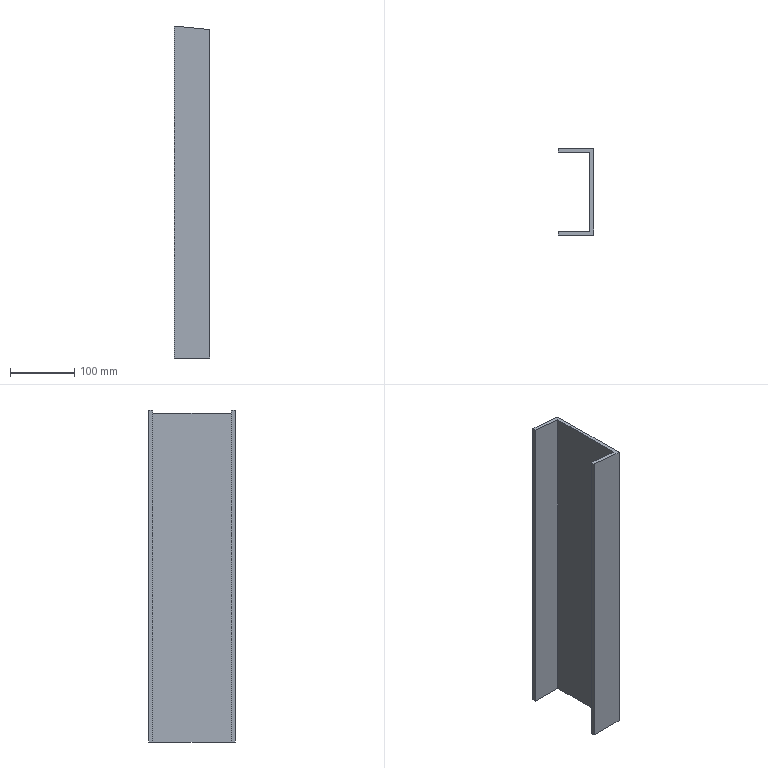Component | NX | LEFT_FRAME600_2 | 1 solid | 10 faces | box 55 x 135 x 517.27 mm | volume 717504 mm3 | plane 10
STEP:
#1=CARTESIAN_POINT('',(0.,0.,0.));
#2=DIRECTION('',(0.,0.,1.));
#3=DIRECTION('',(1.,0.,0.));
#4=AXIS2_PLACEMENT_3D('',#1,#2,#3);
#5=CARTESIAN_POINT('',(55.,0.,511.782));
#6=VERTEX_POINT('',#5);
#7=CARTESIAN_POINT('',(55.,135.,511.782));
#8=VERTEX_POINT('',#7);
#9=CARTESIAN_POINT('',(55.,135.,511.782));
#10=DIRECTION('',(0.,1.,-0.));
#11=VECTOR('',#10,1.);
#12=LINE('',#9,#11);
#13=CARTESIAN_POINT('',(55.,135.,530.));
#14=DIRECTION('',(1.,-0.,0.));
#15=DIRECTION('',(0.,1.,0.));
#16=AXIS2_PLACEMENT_3D('',#13,#14,#15);
#17=PLANE('',#16);
#18=CARTESIAN_POINT('',(0.,-18.218));
#19=DIRECTION('',(1.,-0.));
#20=VECTOR('',#19,1.);
#21=LINE('',#18,#20);
#22=(GEOMETRIC_REPRESENTATION_CONTEXT(2)PARAMETRIC_REPRESENTATION_CONTEXT()REPRESENTATION_CONTEXT('',''));
#23=DEFINITIONAL_REPRESENTATION('',(#21),#22);
#24=PCURVE('',#17,#23);
#25=CARTESIAN_POINT('',(96.917,-235.,507.598));
#26=DIRECTION('',(-0.09932,0.,-0.9951));
#27=DIRECTION('',(0.9951,0.,-0.09932));
#28=AXIS2_PLACEMENT_3D('',#25,#26,#27);
#29=PLANE('',#28);
#30=CARTESIAN_POINT('',(-42.125,-370.));
#31=DIRECTION('',(0.,-1.));
#32=VECTOR('',#31,1.);
#33=LINE('',#30,#32);
#34=(GEOMETRIC_REPRESENTATION_CONTEXT(2)PARAMETRIC_REPRESENTATION_CONTEXT()REPRESENTATION_CONTEXT('',''));
#35=DEFINITIONAL_REPRESENTATION('',(#33),#34);
#36=PCURVE('',#29,#35);
#37=SURFACE_CURVE('',#12,(#24,#36),.PCURVE_S1.);
#38=EDGE_CURVE('',#6,#8,#37,.T.);
#39=ORIENTED_EDGE('',*,*,#38,.F.);
#40=CARTESIAN_POINT('',(55.,0.,0.));
#41=VERTEX_POINT('',#40);
#42=CARTESIAN_POINT('',(55.,0.,530.));
#43=DIRECTION('',(0.,0.,-1.));
#44=VECTOR('',#43,1.);
#45=LINE('',#42,#44);
#46=CARTESIAN_POINT('',(-135.,0.));
#47=DIRECTION('',(0.,-1.));
#48=VECTOR('',#47,1.);
#49=LINE('',#46,#48);
#50=(GEOMETRIC_REPRESENTATION_CONTEXT(2)PARAMETRIC_REPRESENTATION_CONTEXT()REPRESENTATION_CONTEXT('',''));
#51=DEFINITIONAL_REPRESENTATION('',(#49),#50);
#52=PCURVE('',#17,#51);
#53=CARTESIAN_POINT('',(55.,0.,530.));
#54=DIRECTION('',(0.,-1.,0.));
#55=DIRECTION('',(0.,0.,1.));
#56=AXIS2_PLACEMENT_3D('',#53,#54,#55);
#57=PLANE('',#56);
#58=CARTESIAN_POINT('',(0.,0.));
#59=DIRECTION('',(-1.,0.));
#60=VECTOR('',#59,1.);
#61=LINE('',#58,#60);
#62=(GEOMETRIC_REPRESENTATION_CONTEXT(2)PARAMETRIC_REPRESENTATION_CONTEXT()REPRESENTATION_CONTEXT('',''));
#63=DEFINITIONAL_REPRESENTATION('',(#61),#62);
#64=PCURVE('',#57,#63);
#65=SURFACE_CURVE('',#45,(#52,#64),.PCURVE_S1.);
#66=EDGE_CURVE('',#6,#41,#65,.T.);
#67=ORIENTED_EDGE('',*,*,#66,.T.);
#68=CARTESIAN_POINT('',(55.,135.,0.));
#69=VERTEX_POINT('',#68);
#70=CARTESIAN_POINT('',(55.,135.,0.));
#71=DIRECTION('',(-0.,-1.,0.));
#72=VECTOR('',#71,1.);
#73=LINE('',#70,#72);
#74=CARTESIAN_POINT('',(0.,-530.));
#75=DIRECTION('',(-1.,0.));
#76=VECTOR('',#75,1.);
#77=LINE('',#74,#76);
#78=(GEOMETRIC_REPRESENTATION_CONTEXT(2)PARAMETRIC_REPRESENTATION_CONTEXT()REPRESENTATION_CONTEXT('',''));
#79=DEFINITIONAL_REPRESENTATION('',(#77),#78);
#80=PCURVE('',#17,#79);
#81=CARTESIAN_POINT('',(55.,0.,0.));
#82=DIRECTION('',(0.,0.,-1.));
#83=DIRECTION('',(1.,0.,0.));
#84=AXIS2_PLACEMENT_3D('',#81,#82,#83);
#85=PLANE('',#84);
#86=CARTESIAN_POINT('',(0.,-135.));
#87=DIRECTION('',(-0.,1.));
#88=VECTOR('',#87,1.);
#89=LINE('',#86,#88);
#90=(GEOMETRIC_REPRESENTATION_CONTEXT(2)PARAMETRIC_REPRESENTATION_CONTEXT()REPRESENTATION_CONTEXT('',''));
#91=DEFINITIONAL_REPRESENTATION('',(#89),#90);
#92=PCURVE('',#85,#91);
#93=SURFACE_CURVE('',#73,(#80,#92),.PCURVE_S1.);
#94=EDGE_CURVE('',#69,#41,#93,.T.);
#95=ORIENTED_EDGE('',*,*,#94,.F.);
#96=CARTESIAN_POINT('',(55.,135.,530.));
#97=DIRECTION('',(0.,0.,-1.));
#98=VECTOR('',#97,1.);
#99=LINE('',#96,#98);
#100=CARTESIAN_POINT('',(0.,0.));
#101=DIRECTION('',(0.,-1.));
#102=VECTOR('',#101,1.);
#103=LINE('',#100,#102);
#104=(GEOMETRIC_REPRESENTATION_CONTEXT(2)PARAMETRIC_REPRESENTATION_CONTEXT()REPRESENTATION_CONTEXT('',''));
#105=DEFINITIONAL_REPRESENTATION('',(#103),#104);
#106=PCURVE('',#17,#105);
#107=CARTESIAN_POINT('',(0.,135.,530.));
#108=DIRECTION('',(0.,1.,0.));
#109=DIRECTION('',(0.,0.,-1.));
#110=AXIS2_PLACEMENT_3D('',#107,#108,#109);
#111=PLANE('',#110);
#112=CARTESIAN_POINT('',(0.,-55.));
#113=DIRECTION('',(1.,0.));
#114=VECTOR('',#113,1.);
#115=LINE('',#112,#114);
#116=(GEOMETRIC_REPRESENTATION_CONTEXT(2)PARAMETRIC_REPRESENTATION_CONTEXT()REPRESENTATION_CONTEXT('',''));
#117=DEFINITIONAL_REPRESENTATION('',(#115),#116);
#118=PCURVE('',#111,#117);
#119=SURFACE_CURVE('',#99,(#106,#118),.PCURVE_S1.);
#120=EDGE_CURVE('',#8,#69,#119,.T.);
#121=ORIENTED_EDGE('',*,*,#120,.F.);
#122=EDGE_LOOP('',(#39,#67,#95,#121));
#123=FACE_BOUND('',#122,.T.);
#124=ADVANCED_FACE('',(#123),#17,.T.);
#125=CARTESIAN_POINT('',(0.,0.,517.272));
#126=VERTEX_POINT('',#125);
#127=CARTESIAN_POINT('',(53.2,0.,511.962));
#128=DIRECTION('',(0.9951,0.,-0.09932));
#129=VECTOR('',#128,1.);
#130=LINE('',#127,#129);
#131=CARTESIAN_POINT('',(-18.038,1.8));
#132=DIRECTION('',(-0.09932,-0.9951));
#133=VECTOR('',#132,1.);
#134=LINE('',#131,#133);
#135=(GEOMETRIC_REPRESENTATION_CONTEXT(2)PARAMETRIC_REPRESENTATION_CONTEXT()REPRESENTATION_CONTEXT('',''));
#136=DEFINITIONAL_REPRESENTATION('',(#134),#135);
#137=PCURVE('',#57,#136);
#138=CARTESIAN_POINT('',(-43.934,-235.));
#139=DIRECTION('',(1.,0.));
#140=VECTOR('',#139,1.);
#141=LINE('',#138,#140);
#142=(GEOMETRIC_REPRESENTATION_CONTEXT(2)PARAMETRIC_REPRESENTATION_CONTEXT()REPRESENTATION_CONTEXT('',''));
#143=DEFINITIONAL_REPRESENTATION('',(#141),#142);
#144=PCURVE('',#29,#143);
#145=SURFACE_CURVE('',#130,(#137,#144),.PCURVE_S1.);
#146=EDGE_CURVE('',#126,#6,#145,.T.);
#147=ORIENTED_EDGE('',*,*,#146,.F.);
#148=CARTESIAN_POINT('',(0.,0.,0.));
#149=VERTEX_POINT('',#148);
#150=CARTESIAN_POINT('',(0.,0.,530.));
#151=DIRECTION('',(0.,0.,-1.));
#152=VECTOR('',#151,1.);
#153=LINE('',#150,#152);
#154=CARTESIAN_POINT('',(0.,55.));
#155=DIRECTION('',(-1.,0.));
#156=VECTOR('',#155,1.);
#157=LINE('',#154,#156);
#158=(GEOMETRIC_REPRESENTATION_CONTEXT(2)PARAMETRIC_REPRESENTATION_CONTEXT()REPRESENTATION_CONTEXT('',''));
#159=DEFINITIONAL_REPRESENTATION('',(#157),#158);
#160=PCURVE('',#57,#159);
#161=CARTESIAN_POINT('',(0.,0.,530.));
#162=DIRECTION('',(-1.,0.,0.));
#163=DIRECTION('',(-0.,-1.,0.));
#164=AXIS2_PLACEMENT_3D('',#161,#162,#163);
#165=PLANE('',#164);
#166=CARTESIAN_POINT('',(0.,0.));
#167=DIRECTION('',(0.,-1.));
#168=VECTOR('',#167,1.);
#169=LINE('',#166,#168);
#170=(GEOMETRIC_REPRESENTATION_CONTEXT(2)PARAMETRIC_REPRESENTATION_CONTEXT()REPRESENTATION_CONTEXT('',''));
#171=DEFINITIONAL_REPRESENTATION('',(#169),#170);
#172=PCURVE('',#165,#171);
#173=SURFACE_CURVE('',#153,(#160,#172),.PCURVE_S1.);
#174=EDGE_CURVE('',#126,#149,#173,.T.);
#175=ORIENTED_EDGE('',*,*,#174,.T.);
#176=CARTESIAN_POINT('',(55.,0.,0.));
#177=DIRECTION('',(-1.,0.,0.));
#178=VECTOR('',#177,1.);
#179=LINE('',#176,#178);
#180=CARTESIAN_POINT('',(-530.,0.));
#181=DIRECTION('',(0.,1.));
#182=VECTOR('',#181,1.);
#183=LINE('',#180,#182);
#184=(GEOMETRIC_REPRESENTATION_CONTEXT(2)PARAMETRIC_REPRESENTATION_CONTEXT()REPRESENTATION_CONTEXT('',''));
#185=DEFINITIONAL_REPRESENTATION('',(#183),#184);
#186=PCURVE('',#57,#185);
#187=CARTESIAN_POINT('',(0.,0.));
#188=DIRECTION('',(-1.,0.));
#189=VECTOR('',#188,1.);
#190=LINE('',#187,#189);
#191=(GEOMETRIC_REPRESENTATION_CONTEXT(2)PARAMETRIC_REPRESENTATION_CONTEXT()REPRESENTATION_CONTEXT('',''));
#192=DEFINITIONAL_REPRESENTATION('',(#190),#191);
#193=PCURVE('',#85,#192);
#194=SURFACE_CURVE('',#179,(#186,#193),.PCURVE_S1.);
#195=EDGE_CURVE('',#41,#149,#194,.T.);
#196=ORIENTED_EDGE('',*,*,#195,.F.);
#197=ORIENTED_EDGE('',*,*,#66,.F.);
#198=EDGE_LOOP('',(#147,#175,#196,#197));
#199=FACE_BOUND('',#198,.T.);
#200=ADVANCED_FACE('',(#199),#57,.T.);
#201=CARTESIAN_POINT('',(0.,6.,517.272));
#202=VERTEX_POINT('',#201);
#203=CARTESIAN_POINT('',(0.,0.,517.272));
#204=DIRECTION('',(-0.,-1.,0.));
#205=VECTOR('',#204,1.);
#206=LINE('',#203,#205);
#207=CARTESIAN_POINT('',(0.,-12.728));
#208=DIRECTION('',(1.,0.));
#209=VECTOR('',#208,1.);
#210=LINE('',#207,#209);
#211=(GEOMETRIC_REPRESENTATION_CONTEXT(2)PARAMETRIC_REPRESENTATION_CONTEXT()REPRESENTATION_CONTEXT('',''));
#212=DEFINITIONAL_REPRESENTATION('',(#210),#211);
#213=PCURVE('',#165,#212);
#214=CARTESIAN_POINT('',(-97.398,-235.));
#215=DIRECTION('',(-0.,1.));
#216=VECTOR('',#215,1.);
#217=LINE('',#214,#216);
#218=(GEOMETRIC_REPRESENTATION_CONTEXT(2)PARAMETRIC_REPRESENTATION_CONTEXT()REPRESENTATION_CONTEXT('',''));
#219=DEFINITIONAL_REPRESENTATION('',(#217),#218);
#220=PCURVE('',#29,#219);
#221=SURFACE_CURVE('',#206,(#213,#220),.PCURVE_S1.);
#222=EDGE_CURVE('',#202,#126,#221,.T.);
#223=ORIENTED_EDGE('',*,*,#222,.F.);
#224=CARTESIAN_POINT('',(0.,6.,0.));
#225=VERTEX_POINT('',#224);
#226=CARTESIAN_POINT('',(0.,6.,530.));
#227=DIRECTION('',(0.,0.,-1.));
#228=VECTOR('',#227,1.);
#229=LINE('',#226,#228);
#230=CARTESIAN_POINT('',(-6.,0.));
#231=DIRECTION('',(0.,-1.));
#232=VECTOR('',#231,1.);
#233=LINE('',#230,#232);
#234=(GEOMETRIC_REPRESENTATION_CONTEXT(2)PARAMETRIC_REPRESENTATION_CONTEXT()REPRESENTATION_CONTEXT('',''));
#235=DEFINITIONAL_REPRESENTATION('',(#233),#234);
#236=PCURVE('',#165,#235);
#237=CARTESIAN_POINT('',(0.,6.,530.));
#238=DIRECTION('',(0.,1.,0.));
#239=DIRECTION('',(-1.,0.,0.));
#240=AXIS2_PLACEMENT_3D('',#237,#238,#239);
#241=PLANE('',#240);
#242=CARTESIAN_POINT('',(0.,0.));
#243=DIRECTION('',(0.,-1.));
#244=VECTOR('',#243,1.);
#245=LINE('',#242,#244);
#246=(GEOMETRIC_REPRESENTATION_CONTEXT(2)PARAMETRIC_REPRESENTATION_CONTEXT()REPRESENTATION_CONTEXT('',''));
#247=DEFINITIONAL_REPRESENTATION('',(#245),#246);
#248=PCURVE('',#241,#247);
#249=SURFACE_CURVE('',#229,(#236,#248),.PCURVE_S1.);
#250=EDGE_CURVE('',#202,#225,#249,.T.);
#251=ORIENTED_EDGE('',*,*,#250,.T.);
#252=CARTESIAN_POINT('',(0.,0.,0.));
#253=DIRECTION('',(0.,1.,0.));
#254=VECTOR('',#253,1.);
#255=LINE('',#252,#254);
#256=CARTESIAN_POINT('',(0.,-530.));
#257=DIRECTION('',(-1.,0.));
#258=VECTOR('',#257,1.);
#259=LINE('',#256,#258);
#260=(GEOMETRIC_REPRESENTATION_CONTEXT(2)PARAMETRIC_REPRESENTATION_CONTEXT()REPRESENTATION_CONTEXT('',''));
#261=DEFINITIONAL_REPRESENTATION('',(#259),#260);
#262=PCURVE('',#165,#261);
#263=CARTESIAN_POINT('',(-55.,0.));
#264=DIRECTION('',(0.,-1.));
#265=VECTOR('',#264,1.);
#266=LINE('',#263,#265);
#267=(GEOMETRIC_REPRESENTATION_CONTEXT(2)PARAMETRIC_REPRESENTATION_CONTEXT()REPRESENTATION_CONTEXT('',''));
#268=DEFINITIONAL_REPRESENTATION('',(#266),#267);
#269=PCURVE('',#85,#268);
#270=SURFACE_CURVE('',#255,(#262,#269),.PCURVE_S1.);
#271=EDGE_CURVE('',#149,#225,#270,.T.);
#272=ORIENTED_EDGE('',*,*,#271,.F.);
#273=ORIENTED_EDGE('',*,*,#174,.F.);
#274=EDGE_LOOP('',(#223,#251,#272,#273));
#275=FACE_BOUND('',#274,.T.);
#276=ADVANCED_FACE('',(#275),#165,.T.);
#277=CARTESIAN_POINT('',(49.,6.,512.381));
#278=VERTEX_POINT('',#277);
#279=CARTESIAN_POINT('',(-1.258,6.,517.397));
#280=DIRECTION('',(-0.9951,0.,0.09932));
#281=VECTOR('',#280,1.);
#282=LINE('',#279,#281);
#283=CARTESIAN_POINT('',(1.258,-12.603));
#284=DIRECTION('',(0.9951,0.09932));
#285=VECTOR('',#284,1.);
#286=LINE('',#283,#285);
#287=(GEOMETRIC_REPRESENTATION_CONTEXT(2)PARAMETRIC_REPRESENTATION_CONTEXT()REPRESENTATION_CONTEXT('',''));
#288=DEFINITIONAL_REPRESENTATION('',(#286),#287);
#289=PCURVE('',#241,#288);
#290=CARTESIAN_POINT('',(-98.662,-241.));
#291=DIRECTION('',(-1.,-0.));
#292=VECTOR('',#291,1.);
#293=LINE('',#290,#292);
#294=(GEOMETRIC_REPRESENTATION_CONTEXT(2)PARAMETRIC_REPRESENTATION_CONTEXT()REPRESENTATION_CONTEXT('',''));
#295=DEFINITIONAL_REPRESENTATION('',(#293),#294);
#296=PCURVE('',#29,#295);
#297=SURFACE_CURVE('',#282,(#289,#296),.PCURVE_S1.);
#298=EDGE_CURVE('',#278,#202,#297,.T.);
#299=ORIENTED_EDGE('',*,*,#298,.F.);
#300=CARTESIAN_POINT('',(49.,6.,0.));
#301=VERTEX_POINT('',#300);
#302=CARTESIAN_POINT('',(49.,6.,530.));
#303=DIRECTION('',(0.,0.,-1.));
#304=VECTOR('',#303,1.);
#305=LINE('',#302,#304);
#306=CARTESIAN_POINT('',(-49.,0.));
#307=DIRECTION('',(0.,-1.));
#308=VECTOR('',#307,1.);
#309=LINE('',#306,#308);
#310=(GEOMETRIC_REPRESENTATION_CONTEXT(2)PARAMETRIC_REPRESENTATION_CONTEXT()REPRESENTATION_CONTEXT('',''));
#311=DEFINITIONAL_REPRESENTATION('',(#309),#310);
#312=PCURVE('',#241,#311);
#313=CARTESIAN_POINT('',(49.,6.,530.));
#314=DIRECTION('',(-1.,0.,0.));
#315=DIRECTION('',(-0.,-1.,0.));
#316=AXIS2_PLACEMENT_3D('',#313,#314,#315);
#317=PLANE('',#316);
#318=CARTESIAN_POINT('',(0.,0.));
#319=DIRECTION('',(0.,-1.));
#320=VECTOR('',#319,1.);
#321=LINE('',#318,#320);
#322=(GEOMETRIC_REPRESENTATION_CONTEXT(2)PARAMETRIC_REPRESENTATION_CONTEXT()REPRESENTATION_CONTEXT('',''));
#323=DEFINITIONAL_REPRESENTATION('',(#321),#322);
#324=PCURVE('',#317,#323);
#325=SURFACE_CURVE('',#305,(#312,#324),.PCURVE_S1.);
#326=EDGE_CURVE('',#278,#301,#325,.T.);
#327=ORIENTED_EDGE('',*,*,#326,.T.);
#328=CARTESIAN_POINT('',(0.,6.,0.));
#329=DIRECTION('',(1.,-0.,0.));
#330=VECTOR('',#329,1.);
#331=LINE('',#328,#330);
#332=CARTESIAN_POINT('',(0.,-530.));
#333=DIRECTION('',(-1.,0.));
#334=VECTOR('',#333,1.);
#335=LINE('',#332,#334);
#336=(GEOMETRIC_REPRESENTATION_CONTEXT(2)PARAMETRIC_REPRESENTATION_CONTEXT()REPRESENTATION_CONTEXT('',''));
#337=DEFINITIONAL_REPRESENTATION('',(#335),#336);
#338=PCURVE('',#241,#337);
#339=CARTESIAN_POINT('',(-55.,-6.));
#340=DIRECTION('',(1.,0.));
#341=VECTOR('',#340,1.);
#342=LINE('',#339,#341);
#343=(GEOMETRIC_REPRESENTATION_CONTEXT(2)PARAMETRIC_REPRESENTATION_CONTEXT()REPRESENTATION_CONTEXT('',''));
#344=DEFINITIONAL_REPRESENTATION('',(#342),#343);
#345=PCURVE('',#85,#344);
#346=SURFACE_CURVE('',#331,(#338,#345),.PCURVE_S1.);
#347=EDGE_CURVE('',#225,#301,#346,.T.);
#348=ORIENTED_EDGE('',*,*,#347,.F.);
#349=ORIENTED_EDGE('',*,*,#250,.F.);
#350=EDGE_LOOP('',(#299,#327,#348,#349));
#351=FACE_BOUND('',#350,.T.);
#352=ADVANCED_FACE('',(#351),#241,.T.);
#353=CARTESIAN_POINT('',(49.,129.,512.381));
#354=VERTEX_POINT('',#353);
#355=CARTESIAN_POINT('',(49.,6.,512.381));
#356=DIRECTION('',(-0.,-1.,0.));
#357=VECTOR('',#356,1.);
#358=LINE('',#355,#357);
#359=CARTESIAN_POINT('',(0.,-17.619));
#360=DIRECTION('',(1.,0.));
#361=VECTOR('',#360,1.);
#362=LINE('',#359,#361);
#363=(GEOMETRIC_REPRESENTATION_CONTEXT(2)PARAMETRIC_REPRESENTATION_CONTEXT()REPRESENTATION_CONTEXT('',''));
#364=DEFINITIONAL_REPRESENTATION('',(#362),#363);
#365=PCURVE('',#317,#364);
#366=CARTESIAN_POINT('',(-48.155,-241.));
#367=DIRECTION('',(-0.,1.));
#368=VECTOR('',#367,1.);
#369=LINE('',#366,#368);
#370=(GEOMETRIC_REPRESENTATION_CONTEXT(2)PARAMETRIC_REPRESENTATION_CONTEXT()REPRESENTATION_CONTEXT('',''));
#371=DEFINITIONAL_REPRESENTATION('',(#369),#370);
#372=PCURVE('',#29,#371);
#373=SURFACE_CURVE('',#358,(#365,#372),.PCURVE_S1.);
#374=EDGE_CURVE('',#354,#278,#373,.T.);
#375=ORIENTED_EDGE('',*,*,#374,.F.);
#376=CARTESIAN_POINT('',(49.,129.,0.));
#377=VERTEX_POINT('',#376);
#378=CARTESIAN_POINT('',(49.,129.,530.));
#379=DIRECTION('',(0.,0.,-1.));
#380=VECTOR('',#379,1.);
#381=LINE('',#378,#380);
#382=CARTESIAN_POINT('',(-123.,0.));
#383=DIRECTION('',(0.,-1.));
#384=VECTOR('',#383,1.);
#385=LINE('',#382,#384);
#386=(GEOMETRIC_REPRESENTATION_CONTEXT(2)PARAMETRIC_REPRESENTATION_CONTEXT()REPRESENTATION_CONTEXT('',''));
#387=DEFINITIONAL_REPRESENTATION('',(#385),#386);
#388=PCURVE('',#317,#387);
#389=CARTESIAN_POINT('',(49.,129.,530.));
#390=DIRECTION('',(-0.,-1.,0.));
#391=DIRECTION('',(1.,-0.,0.));
#392=AXIS2_PLACEMENT_3D('',#389,#390,#391);
#393=PLANE('',#392);
#394=CARTESIAN_POINT('',(0.,0.));
#395=DIRECTION('',(0.,-1.));
#396=VECTOR('',#395,1.);
#397=LINE('',#394,#396);
#398=(GEOMETRIC_REPRESENTATION_CONTEXT(2)PARAMETRIC_REPRESENTATION_CONTEXT()REPRESENTATION_CONTEXT('',''));
#399=DEFINITIONAL_REPRESENTATION('',(#397),#398);
#400=PCURVE('',#393,#399);
#401=SURFACE_CURVE('',#381,(#388,#400),.PCURVE_S1.);
#402=EDGE_CURVE('',#354,#377,#401,.T.);
#403=ORIENTED_EDGE('',*,*,#402,.T.);
#404=CARTESIAN_POINT('',(49.,6.,0.));
#405=DIRECTION('',(0.,1.,0.));
#406=VECTOR('',#405,1.);
#407=LINE('',#404,#406);
#408=CARTESIAN_POINT('',(0.,-530.));
#409=DIRECTION('',(-1.,0.));
#410=VECTOR('',#409,1.);
#411=LINE('',#408,#410);
#412=(GEOMETRIC_REPRESENTATION_CONTEXT(2)PARAMETRIC_REPRESENTATION_CONTEXT()REPRESENTATION_CONTEXT('',''));
#413=DEFINITIONAL_REPRESENTATION('',(#411),#412);
#414=PCURVE('',#317,#413);
#415=CARTESIAN_POINT('',(-6.,-6.));
#416=DIRECTION('',(0.,-1.));
#417=VECTOR('',#416,1.);
#418=LINE('',#415,#417);
#419=(GEOMETRIC_REPRESENTATION_CONTEXT(2)PARAMETRIC_REPRESENTATION_CONTEXT()REPRESENTATION_CONTEXT('',''));
#420=DEFINITIONAL_REPRESENTATION('',(#418),#419);
#421=PCURVE('',#85,#420);
#422=SURFACE_CURVE('',#407,(#414,#421),.PCURVE_S1.);
#423=EDGE_CURVE('',#301,#377,#422,.T.);
#424=ORIENTED_EDGE('',*,*,#423,.F.);
#425=ORIENTED_EDGE('',*,*,#326,.F.);
#426=EDGE_LOOP('',(#375,#403,#424,#425));
#427=FACE_BOUND('',#426,.T.);
#428=ADVANCED_FACE('',(#427),#317,.T.);
#429=CARTESIAN_POINT('',(0.,129.,517.272));
#430=VERTEX_POINT('',#429);
#431=CARTESIAN_POINT('',(47.259,129.,512.555));
#432=DIRECTION('',(0.9951,-0.,-0.09932));
#433=VECTOR('',#432,1.);
#434=LINE('',#431,#433);
#435=CARTESIAN_POINT('',(-1.741,-17.445));
#436=DIRECTION('',(0.9951,-0.09932));
#437=VECTOR('',#436,1.);
#438=LINE('',#435,#437);
#439=(GEOMETRIC_REPRESENTATION_CONTEXT(2)PARAMETRIC_REPRESENTATION_CONTEXT()REPRESENTATION_CONTEXT('',''));
#440=DEFINITIONAL_REPRESENTATION('',(#438),#439);
#441=PCURVE('',#393,#440);
#442=CARTESIAN_POINT('',(-49.905,-364.));
#443=DIRECTION('',(1.,0.));
#444=VECTOR('',#443,1.);
#445=LINE('',#442,#444);
#446=(GEOMETRIC_REPRESENTATION_CONTEXT(2)PARAMETRIC_REPRESENTATION_CONTEXT()REPRESENTATION_CONTEXT('',''));
#447=DEFINITIONAL_REPRESENTATION('',(#445),#446);
#448=PCURVE('',#29,#447);
#449=SURFACE_CURVE('',#434,(#441,#448),.PCURVE_S1.);
#450=EDGE_CURVE('',#430,#354,#449,.T.);
#451=ORIENTED_EDGE('',*,*,#450,.F.);
#452=CARTESIAN_POINT('',(0.,129.,0.));
#453=VERTEX_POINT('',#452);
#454=CARTESIAN_POINT('',(0.,129.,530.));
#455=DIRECTION('',(0.,0.,-1.));
#456=VECTOR('',#455,1.);
#457=LINE('',#454,#456);
#458=CARTESIAN_POINT('',(-49.,0.));
#459=DIRECTION('',(0.,-1.));
#460=VECTOR('',#459,1.);
#461=LINE('',#458,#460);
#462=(GEOMETRIC_REPRESENTATION_CONTEXT(2)PARAMETRIC_REPRESENTATION_CONTEXT()REPRESENTATION_CONTEXT('',''));
#463=DEFINITIONAL_REPRESENTATION('',(#461),#462);
#464=PCURVE('',#393,#463);
#465=CARTESIAN_POINT('',(0.,129.,530.));
#466=DIRECTION('',(-1.,0.,0.));
#467=DIRECTION('',(0.,0.,-1.));
#468=AXIS2_PLACEMENT_3D('',#465,#466,#467);
#469=PLANE('',#468);
#470=CARTESIAN_POINT('',(0.,0.));
#471=DIRECTION('',(1.,0.));
#472=VECTOR('',#471,1.);
#473=LINE('',#470,#472);
#474=(GEOMETRIC_REPRESENTATION_CONTEXT(2)PARAMETRIC_REPRESENTATION_CONTEXT()REPRESENTATION_CONTEXT('',''));
#475=DEFINITIONAL_REPRESENTATION('',(#473),#474);
#476=PCURVE('',#469,#475);
#477=SURFACE_CURVE('',#457,(#464,#476),.PCURVE_S1.);
#478=EDGE_CURVE('',#430,#453,#477,.T.);
#479=ORIENTED_EDGE('',*,*,#478,.T.);
#480=CARTESIAN_POINT('',(49.,129.,0.));
#481=DIRECTION('',(-1.,0.,0.));
#482=VECTOR('',#481,1.);
#483=LINE('',#480,#482);
#484=CARTESIAN_POINT('',(0.,-530.));
#485=DIRECTION('',(-1.,0.));
#486=VECTOR('',#485,1.);
#487=LINE('',#484,#486);
#488=(GEOMETRIC_REPRESENTATION_CONTEXT(2)PARAMETRIC_REPRESENTATION_CONTEXT()REPRESENTATION_CONTEXT('',''));
#489=DEFINITIONAL_REPRESENTATION('',(#487),#488);
#490=PCURVE('',#393,#489);
#491=CARTESIAN_POINT('',(-6.,-129.));
#492=DIRECTION('',(-1.,-0.));
#493=VECTOR('',#492,1.);
#494=LINE('',#491,#493);
#495=(GEOMETRIC_REPRESENTATION_CONTEXT(2)PARAMETRIC_REPRESENTATION_CONTEXT()REPRESENTATION_CONTEXT('',''));
#496=DEFINITIONAL_REPRESENTATION('',(#494),#495);
#497=PCURVE('',#85,#496);
#498=SURFACE_CURVE('',#483,(#490,#497),.PCURVE_S1.);
#499=EDGE_CURVE('',#377,#453,#498,.T.);
#500=ORIENTED_EDGE('',*,*,#499,.F.);
#501=ORIENTED_EDGE('',*,*,#402,.F.);
#502=EDGE_LOOP('',(#451,#479,#500,#501));
#503=FACE_BOUND('',#502,.T.);
#504=ADVANCED_FACE('',(#503),#393,.T.);
#505=CARTESIAN_POINT('',(0.,135.,517.272));
#506=VERTEX_POINT('',#505);
#507=CARTESIAN_POINT('',(0.,129.,517.272));
#508=DIRECTION('',(0.,-1.,0.));
#509=VECTOR('',#508,1.);
#510=LINE('',#507,#509);
#511=CARTESIAN_POINT('',(12.728,0.));
#512=DIRECTION('',(0.,1.));
#513=VECTOR('',#512,1.);
#514=LINE('',#511,#513);
#515=(GEOMETRIC_REPRESENTATION_CONTEXT(2)PARAMETRIC_REPRESENTATION_CONTEXT()REPRESENTATION_CONTEXT('',''));
#516=DEFINITIONAL_REPRESENTATION('',(#514),#515);
#517=PCURVE('',#469,#516);
#518=CARTESIAN_POINT('',(-97.398,-364.));
#519=DIRECTION('',(0.,1.));
#520=VECTOR('',#519,1.);
#521=LINE('',#518,#520);
#522=(GEOMETRIC_REPRESENTATION_CONTEXT(2)PARAMETRIC_REPRESENTATION_CONTEXT()REPRESENTATION_CONTEXT('',''));
#523=DEFINITIONAL_REPRESENTATION('',(#521),#522);
#524=PCURVE('',#29,#523);
#525=SURFACE_CURVE('',#510,(#517,#524),.PCURVE_S1.);
#526=EDGE_CURVE('',#506,#430,#525,.T.);
#527=ORIENTED_EDGE('',*,*,#526,.F.);
#528=CARTESIAN_POINT('',(0.,135.,0.));
#529=VERTEX_POINT('',#528);
#530=CARTESIAN_POINT('',(0.,135.,530.));
#531=DIRECTION('',(0.,0.,-1.));
#532=VECTOR('',#531,1.);
#533=LINE('',#530,#532);
#534=CARTESIAN_POINT('',(0.,-6.));
#535=DIRECTION('',(1.,0.));
#536=VECTOR('',#535,1.);
#537=LINE('',#534,#536);
#538=(GEOMETRIC_REPRESENTATION_CONTEXT(2)PARAMETRIC_REPRESENTATION_CONTEXT()REPRESENTATION_CONTEXT('',''));
#539=DEFINITIONAL_REPRESENTATION('',(#537),#538);
#540=PCURVE('',#469,#539);
#541=CARTESIAN_POINT('',(0.,0.));
#542=DIRECTION('',(1.,0.));
#543=VECTOR('',#542,1.);
#544=LINE('',#541,#543);
#545=(GEOMETRIC_REPRESENTATION_CONTEXT(2)PARAMETRIC_REPRESENTATION_CONTEXT()REPRESENTATION_CONTEXT('',''));
#546=DEFINITIONAL_REPRESENTATION('',(#544),#545);
#547=PCURVE('',#111,#546);
#548=SURFACE_CURVE('',#533,(#540,#547),.PCURVE_S1.);
#549=EDGE_CURVE('',#506,#529,#548,.T.);
#550=ORIENTED_EDGE('',*,*,#549,.T.);
#551=CARTESIAN_POINT('',(0.,129.,0.));
#552=DIRECTION('',(0.,1.,0.));
#553=VECTOR('',#552,1.);
#554=LINE('',#551,#553);
#555=CARTESIAN_POINT('',(530.,0.));
#556=DIRECTION('',(0.,-1.));
#557=VECTOR('',#556,1.);
#558=LINE('',#555,#557);
#559=(GEOMETRIC_REPRESENTATION_CONTEXT(2)PARAMETRIC_REPRESENTATION_CONTEXT()REPRESENTATION_CONTEXT('',''));
#560=DEFINITIONAL_REPRESENTATION('',(#558),#559);
#561=PCURVE('',#469,#560);
#562=CARTESIAN_POINT('',(-55.,-129.));
#563=DIRECTION('',(0.,-1.));
#564=VECTOR('',#563,1.);
#565=LINE('',#562,#564);
#566=(GEOMETRIC_REPRESENTATION_CONTEXT(2)PARAMETRIC_REPRESENTATION_CONTEXT()REPRESENTATION_CONTEXT('',''));
#567=DEFINITIONAL_REPRESENTATION('',(#565),#566);
#568=PCURVE('',#85,#567);
#569=SURFACE_CURVE('',#554,(#561,#568),.PCURVE_S1.);
#570=EDGE_CURVE('',#453,#529,#569,.T.);
#571=ORIENTED_EDGE('',*,*,#570,.F.);
#572=ORIENTED_EDGE('',*,*,#478,.F.);
#573=EDGE_LOOP('',(#527,#550,#571,#572));
#574=FACE_BOUND('',#573,.T.);
#575=ADVANCED_FACE('',(#574),#469,.T.);
#576=CARTESIAN_POINT('',(96.917,135.,507.598));
#577=DIRECTION('',(-0.9951,0.,0.09932));
#578=VECTOR('',#577,1.);
#579=LINE('',#576,#578);
#580=CARTESIAN_POINT('',(22.402,-96.917));
#581=DIRECTION('',(-0.09932,0.9951));
#582=VECTOR('',#581,1.);
#583=LINE('',#580,#582);
#584=(GEOMETRIC_REPRESENTATION_CONTEXT(2)PARAMETRIC_REPRESENTATION_CONTEXT()REPRESENTATION_CONTEXT('',''));
#585=DEFINITIONAL_REPRESENTATION('',(#583),#584);
#586=PCURVE('',#111,#585);
#587=CARTESIAN_POINT('',(0.,-370.));
#588=DIRECTION('',(-1.,0.));
#589=VECTOR('',#588,1.);
#590=LINE('',#587,#589);
#591=(GEOMETRIC_REPRESENTATION_CONTEXT(2)PARAMETRIC_REPRESENTATION_CONTEXT()REPRESENTATION_CONTEXT('',''));
#592=DEFINITIONAL_REPRESENTATION('',(#590),#591);
#593=PCURVE('',#29,#592);
#594=SURFACE_CURVE('',#579,(#586,#593),.PCURVE_S1.);
#595=EDGE_CURVE('',#8,#506,#594,.T.);
#596=ORIENTED_EDGE('',*,*,#595,.F.);
#597=ORIENTED_EDGE('',*,*,#120,.T.);
#598=CARTESIAN_POINT('',(0.,135.,0.));
#599=DIRECTION('',(1.,0.,0.));
#600=VECTOR('',#599,1.);
#601=LINE('',#598,#600);
#602=CARTESIAN_POINT('',(530.,0.));
#603=DIRECTION('',(0.,-1.));
#604=VECTOR('',#603,1.);
#605=LINE('',#602,#604);
#606=(GEOMETRIC_REPRESENTATION_CONTEXT(2)PARAMETRIC_REPRESENTATION_CONTEXT()REPRESENTATION_CONTEXT('',''));
#607=DEFINITIONAL_REPRESENTATION('',(#605),#606);
#608=PCURVE('',#111,#607);
#609=CARTESIAN_POINT('',(-55.,-135.));
#610=DIRECTION('',(1.,0.));
#611=VECTOR('',#610,1.);
#612=LINE('',#609,#611);
#613=(GEOMETRIC_REPRESENTATION_CONTEXT(2)PARAMETRIC_REPRESENTATION_CONTEXT()REPRESENTATION_CONTEXT('',''));
#614=DEFINITIONAL_REPRESENTATION('',(#612),#613);
#615=PCURVE('',#85,#614);
#616=SURFACE_CURVE('',#601,(#608,#615),.PCURVE_S1.);
#617=EDGE_CURVE('',#529,#69,#616,.T.);
#618=ORIENTED_EDGE('',*,*,#617,.F.);
#619=ORIENTED_EDGE('',*,*,#549,.F.);
#620=EDGE_LOOP('',(#596,#597,#618,#619));
#621=FACE_BOUND('',#620,.T.);
#622=ADVANCED_FACE('',(#621),#111,.T.);
#623=ORIENTED_EDGE('',*,*,#94,.T.);
#624=ORIENTED_EDGE('',*,*,#195,.T.);
#625=ORIENTED_EDGE('',*,*,#271,.T.);
#626=ORIENTED_EDGE('',*,*,#347,.T.);
#627=ORIENTED_EDGE('',*,*,#423,.T.);
#628=ORIENTED_EDGE('',*,*,#499,.T.);
#629=ORIENTED_EDGE('',*,*,#570,.T.);
#630=ORIENTED_EDGE('',*,*,#617,.T.);
#631=EDGE_LOOP('',(#623,#624,#625,#626,#627,#628,#629,#630));
#632=FACE_BOUND('',#631,.T.);
#633=ADVANCED_FACE('',(#632),#85,.T.);
#634=ORIENTED_EDGE('',*,*,#38,.T.);
#635=ORIENTED_EDGE('',*,*,#595,.T.);
#636=ORIENTED_EDGE('',*,*,#526,.T.);
#637=ORIENTED_EDGE('',*,*,#450,.T.);
#638=ORIENTED_EDGE('',*,*,#374,.T.);
#639=ORIENTED_EDGE('',*,*,#298,.T.);
#640=ORIENTED_EDGE('',*,*,#222,.T.);
#641=ORIENTED_EDGE('',*,*,#146,.T.);
#642=EDGE_LOOP('',(#634,#635,#636,#637,#638,#639,#640,#641));
#643=FACE_BOUND('',#642,.T.);
#644=ADVANCED_FACE('',(#643),#29,.F.);
#645=CLOSED_SHELL('',(#124,#200,#276,#352,#428,#504,#575,#622,#633,#644));
#646=MANIFOLD_SOLID_BREP('',#645);
#647=(LENGTH_UNIT()NAMED_UNIT(*)SI_UNIT(.MILLI.,.METRE.));
#648=UNCERTAINTY_MEASURE_WITH_UNIT(LENGTH_MEASURE(0.0000001),#647,'','');
#649=(NAMED_UNIT(*)PLANE_ANGLE_UNIT()SI_UNIT($,.RADIAN.));
#650=(NAMED_UNIT(*)SI_UNIT($,.STERADIAN.)SOLID_ANGLE_UNIT());
#651=(GEOMETRIC_REPRESENTATION_CONTEXT(3)GLOBAL_UNCERTAINTY_ASSIGNED_CONTEXT((#648))GLOBAL_UNIT_ASSIGNED_CONTEXT((#647,#649,#650))REPRESENTATION_CONTEXT('',''));
#652=ADVANCED_BREP_SHAPE_REPRESENTATION('',(#4,#646),#651);